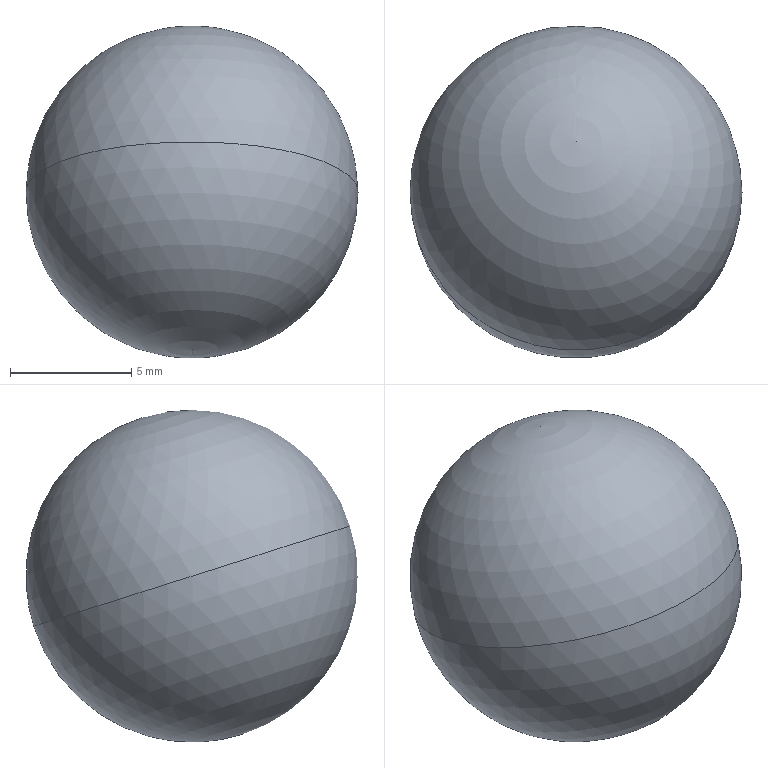Component | SolidWorks | UpperHousingAssembly-1_WormAxisAssembly-1_DeepGrooveBallBearing6309-1_RollingElement-1 | 1 solid | 2 faces | box 13.7 x 13.7 x 13.7 mm | volume 1346 mm3 | sphere 2
build123d program:
from build123d import *


with BuildPart() as part:
    # Sketch1 → Revolve1 (revolve)
    with BuildSketch(Plane.XY):
        with BuildLine():
            Line((29.4, 0), (43.1, 0))
            ThreePointArc((43.1, 0), (36.25, 6.85), (29.4, 0))
        make_face()
    revolve(axis=Axis((0, 0, 0), (1, 0, 0)))


solid = part.part

# Placed as in the assembly
solid = solid.moved(Location((982.827, 1435.618, 1670.06), (0, 0, 0)))
STEP:
#1=COLOUR_RGB('',0.7922,0.8196,0.9333);
#2=FILL_AREA_STYLE_COLOUR('',#1);
#3=FILL_AREA_STYLE('',(#2));
#4=SURFACE_STYLE_FILL_AREA(#3);
#5=SURFACE_SIDE_STYLE('',(#4));
#6=SURFACE_STYLE_USAGE(.BOTH.,#5);
#7=PRESENTATION_STYLE_ASSIGNMENT((#6));
#8=CARTESIAN_POINT('',(40.391,56.52,65.75));
#9=VERTEX_POINT('',#8);
#10=CARTESIAN_POINT('',(39.851,56.52,65.75));
#11=VERTEX_POINT('',#10);
#12=CARTESIAN_POINT('',(40.121,56.52,65.75));
#13=DIRECTION('',(0.,0.3024,0.9532));
#14=DIRECTION('',(0.,-0.9532,0.3024));
#15=AXIS2_PLACEMENT_3D('',#12,#13,#14);
#16=CIRCLE('',#15,0.2697);
#17=EDGE_CURVE('',#9,#11,#16,.T.);
#18=ORIENTED_EDGE('',*,*,#17,.F.);
#19=CARTESIAN_POINT('',(40.121,56.52,65.75));
#20=DIRECTION('',(0.,-0.3024,-0.9532));
#21=DIRECTION('',(0.,0.9532,-0.3024));
#22=AXIS2_PLACEMENT_3D('',#19,#20,#21);
#23=CIRCLE('',#22,0.2697);
#24=EDGE_CURVE('',#9,#11,#23,.T.);
#25=ORIENTED_EDGE('',*,*,#24,.T.);
#26=EDGE_LOOP('',(#18,#25));
#27=FACE_OUTER_BOUND('',#26,.T.);
#28=CARTESIAN_POINT('',(40.121,56.52,65.75));
#29=DIRECTION('',(0.,-0.3024,-0.9532));
#30=DIRECTION('',(0.,0.9532,-0.3024));
#31=AXIS2_PLACEMENT_3D('',#28,#29,#30);
#32=SPHERICAL_SURFACE('',#31,0.2697);
#33=ADVANCED_FACE('',(#27),#32,.T.);
#34=ORIENTED_EDGE('',*,*,#24,.F.);
#35=ORIENTED_EDGE('',*,*,#17,.T.);
#36=EDGE_LOOP('',(#34,#35));
#37=FACE_OUTER_BOUND('',#36,.T.);
#38=CARTESIAN_POINT('',(40.121,56.52,65.75));
#39=DIRECTION('',(0.,-0.3024,-0.9532));
#40=DIRECTION('',(0.,0.9532,-0.3024));
#41=AXIS2_PLACEMENT_3D('',#38,#39,#40);
#42=SPHERICAL_SURFACE('',#41,0.2697);
#43=ADVANCED_FACE('',(#37),#42,.T.);
#44=CLOSED_SHELL('',(#33,#43));
#45=MANIFOLD_SOLID_BREP('',#44);
#46=STYLED_ITEM('',(#7),#45);
#47=(LENGTH_UNIT()NAMED_UNIT(*)SI_UNIT($,.METRE.));
#48=LENGTH_MEASURE_WITH_UNIT(LENGTH_MEASURE(0.0254),#47);
#49=DIMENSIONAL_EXPONENTS(1.,0.,0.,0.,0.,0.,0.);
#50=(CONVERSION_BASED_UNIT('',#48)LENGTH_UNIT()NAMED_UNIT(#49));
#51=UNCERTAINTY_MEASURE_WITH_UNIT(LENGTH_MEASURE(0.00001),#50,'','');
#52=(NAMED_UNIT(*)PLANE_ANGLE_UNIT()SI_UNIT($,.RADIAN.));
#53=(NAMED_UNIT(*)SI_UNIT($,.STERADIAN.)SOLID_ANGLE_UNIT());
#54=(GEOMETRIC_REPRESENTATION_CONTEXT(3)GLOBAL_UNCERTAINTY_ASSIGNED_CONTEXT((#51))GLOBAL_UNIT_ASSIGNED_CONTEXT((#50,#52,#53))REPRESENTATION_CONTEXT('',''));
#55=MECHANICAL_DESIGN_GEOMETRIC_PRESENTATION_REPRESENTATION('',(#46),#54);
#56=CARTESIAN_POINT('',(0.,0.,0.));
#57=DIRECTION('',(0.,0.,1.));
#58=DIRECTION('',(1.,0.,0.));
#59=AXIS2_PLACEMENT_3D('',#56,#57,#58);
#60=(LENGTH_UNIT()NAMED_UNIT(*)SI_UNIT($,.METRE.));
#61=LENGTH_MEASURE_WITH_UNIT(LENGTH_MEASURE(0.0254),#60);
#62=DIMENSIONAL_EXPONENTS(1.,0.,0.,0.,0.,0.,0.);
#63=(CONVERSION_BASED_UNIT('',#61)LENGTH_UNIT()NAMED_UNIT(#62));
#64=UNCERTAINTY_MEASURE_WITH_UNIT(LENGTH_MEASURE(0.00001),#63,'','');
#65=(NAMED_UNIT(*)PLANE_ANGLE_UNIT()SI_UNIT($,.RADIAN.));
#66=(NAMED_UNIT(*)SI_UNIT($,.STERADIAN.)SOLID_ANGLE_UNIT());
#67=(GEOMETRIC_REPRESENTATION_CONTEXT(3)GLOBAL_UNCERTAINTY_ASSIGNED_CONTEXT((#64))GLOBAL_UNIT_ASSIGNED_CONTEXT((#63,#65,#66))REPRESENTATION_CONTEXT('',''));
#68=ADVANCED_BREP_SHAPE_REPRESENTATION('',(#45,#59),#67);
#69=PRESENTATION_LAYER_ASSIGNMENT('','',(#46));